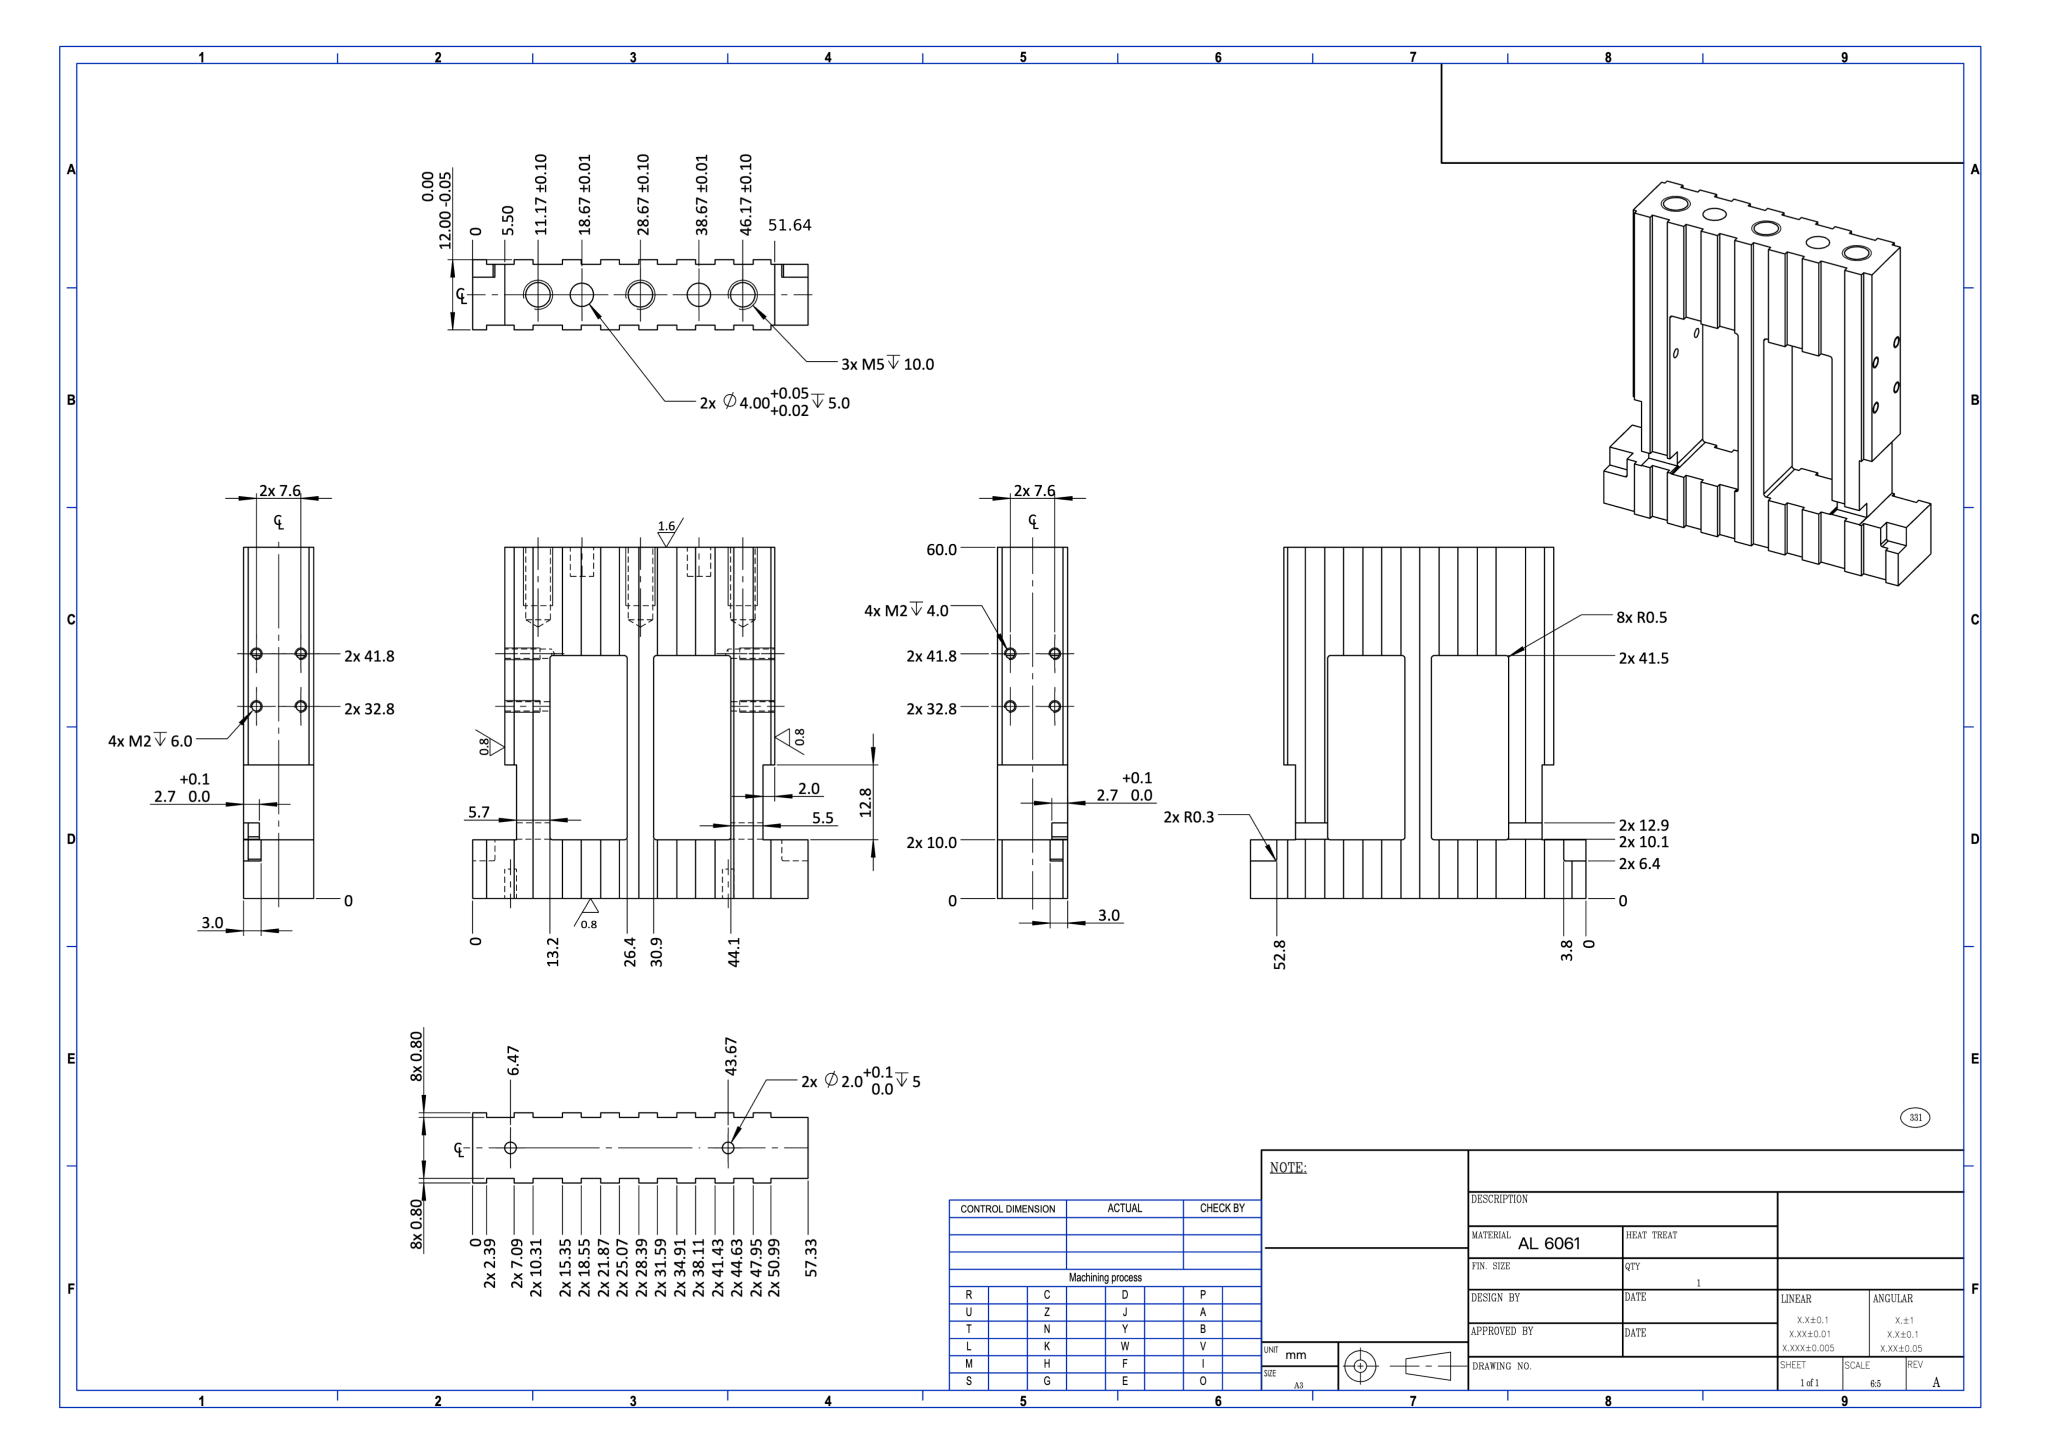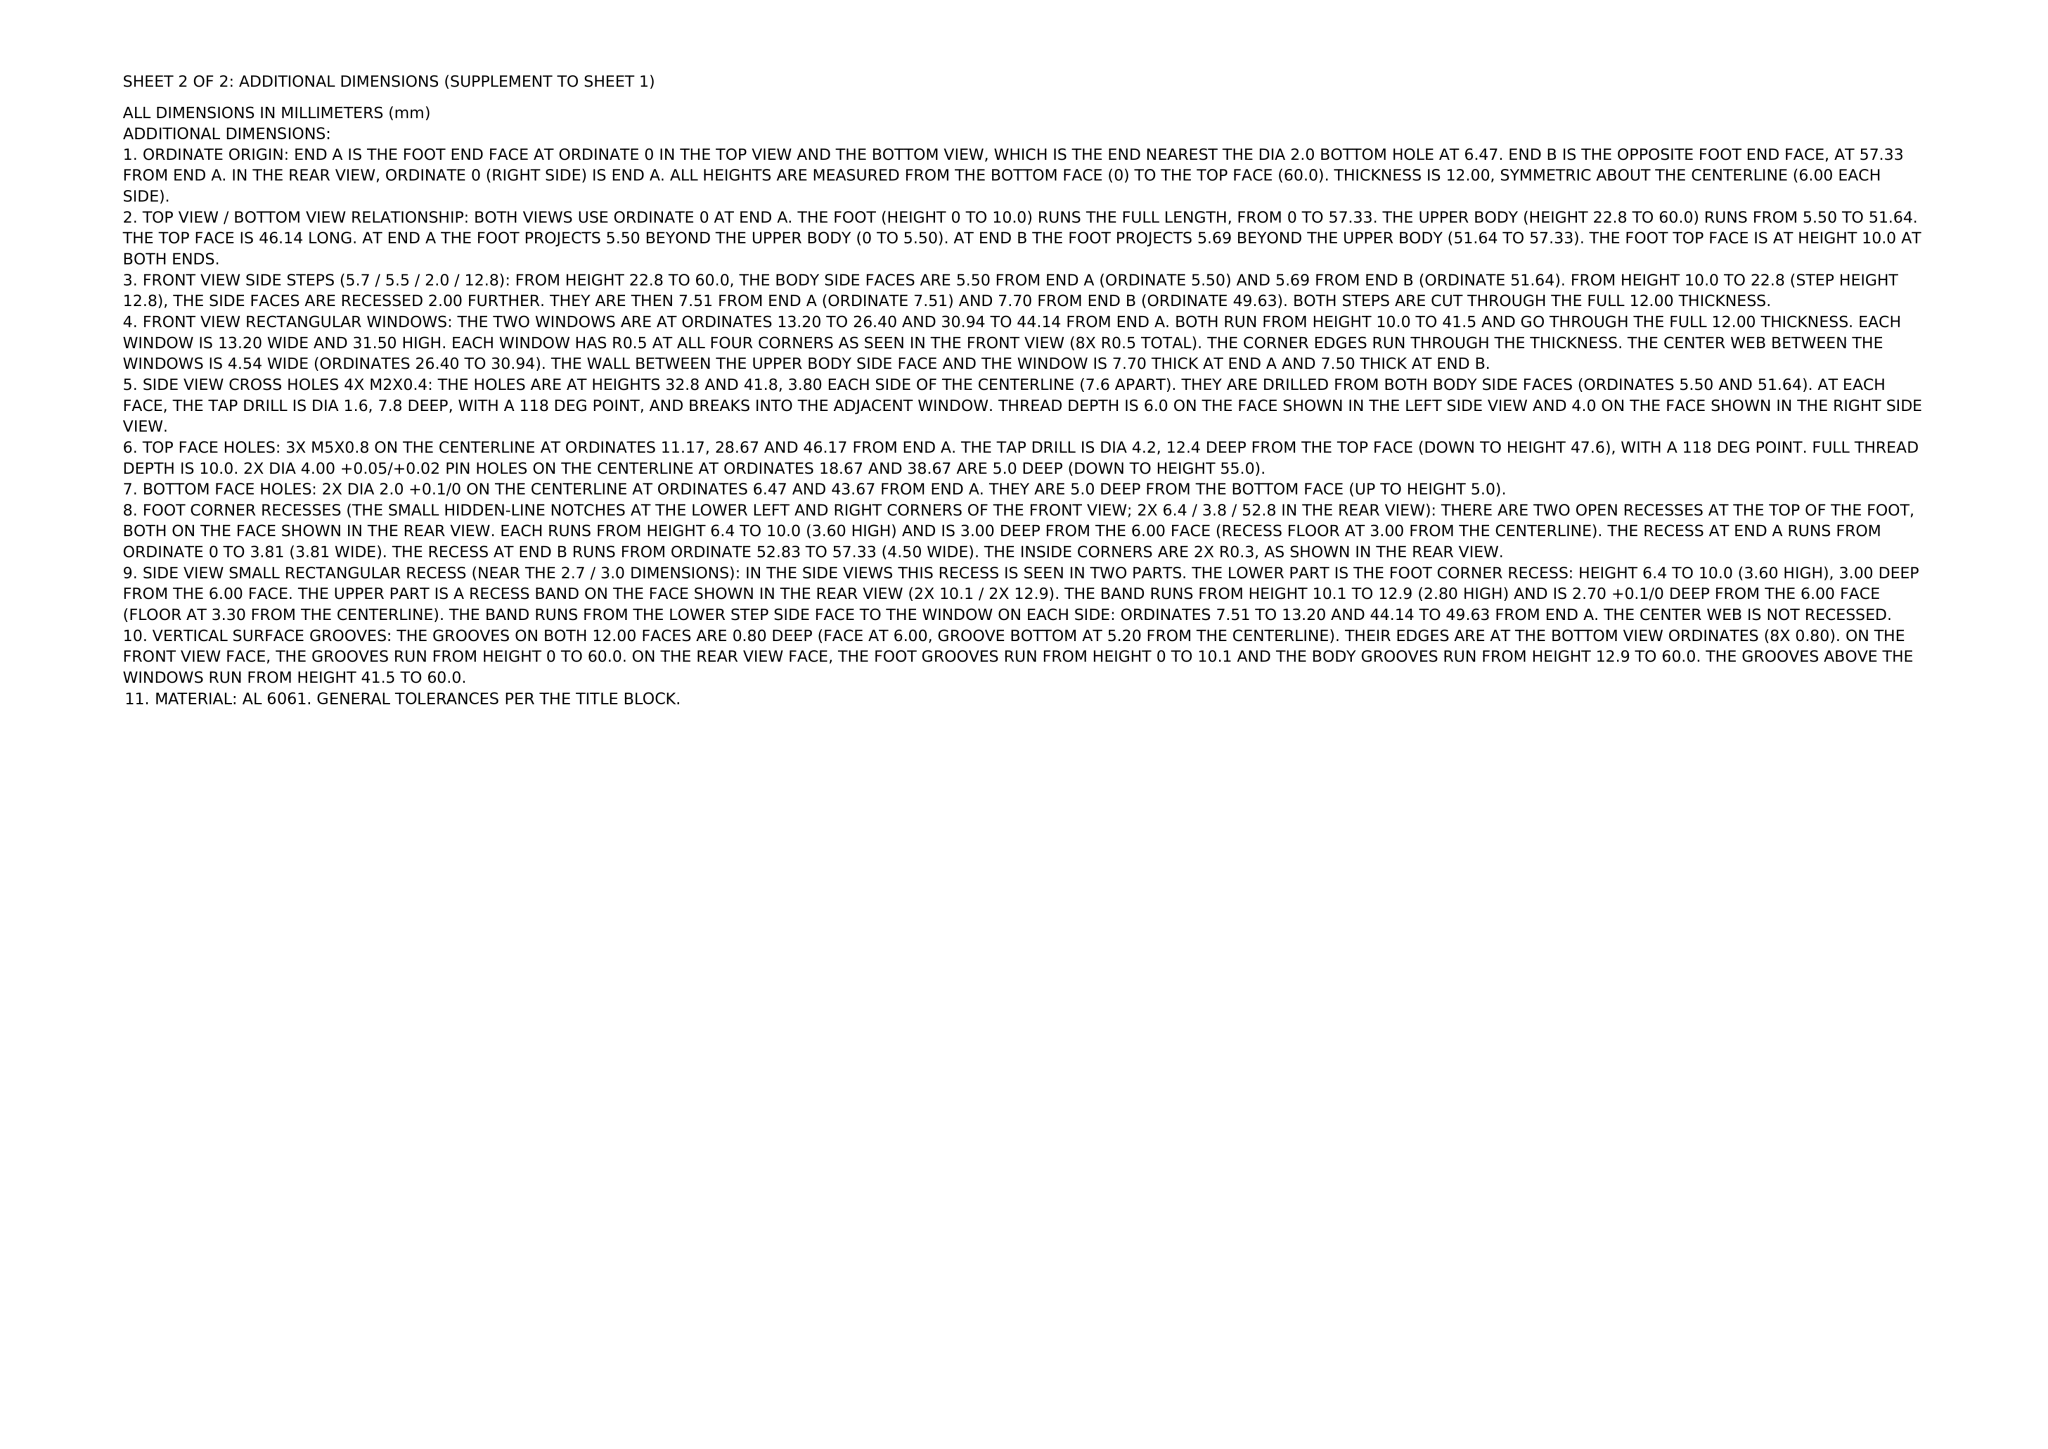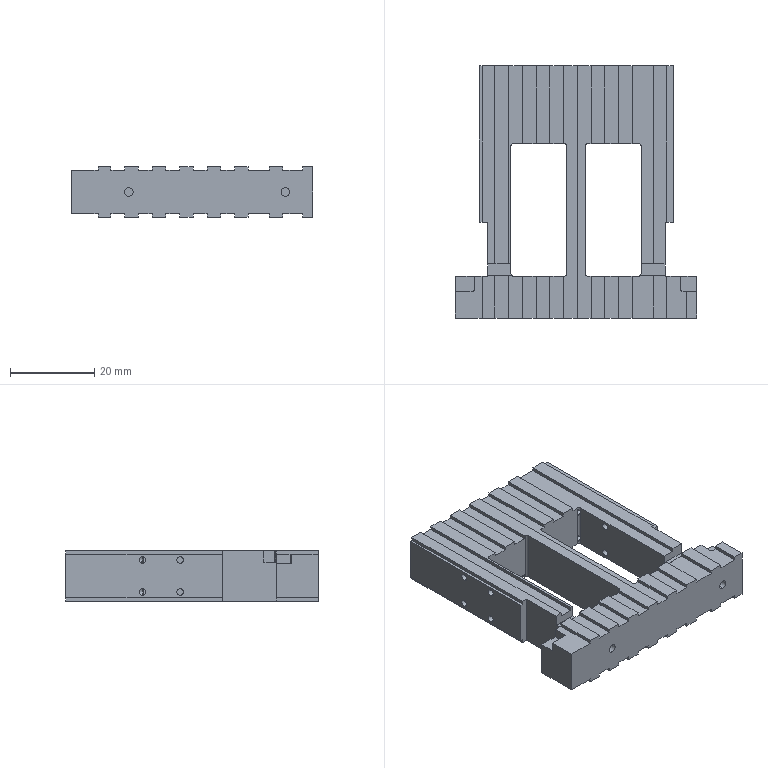Part | NX | mm | 1 solid | 202 faces | box 57.33 x 60 x 12 mm | volume 21300 mm3 | plane 142 | cylinder 46 | cone 14 | commonest cylinder face diameters 1.6 x16 1 x12 4.2 x6 4 x4 2 x4 1.2 x2 0.6 x2